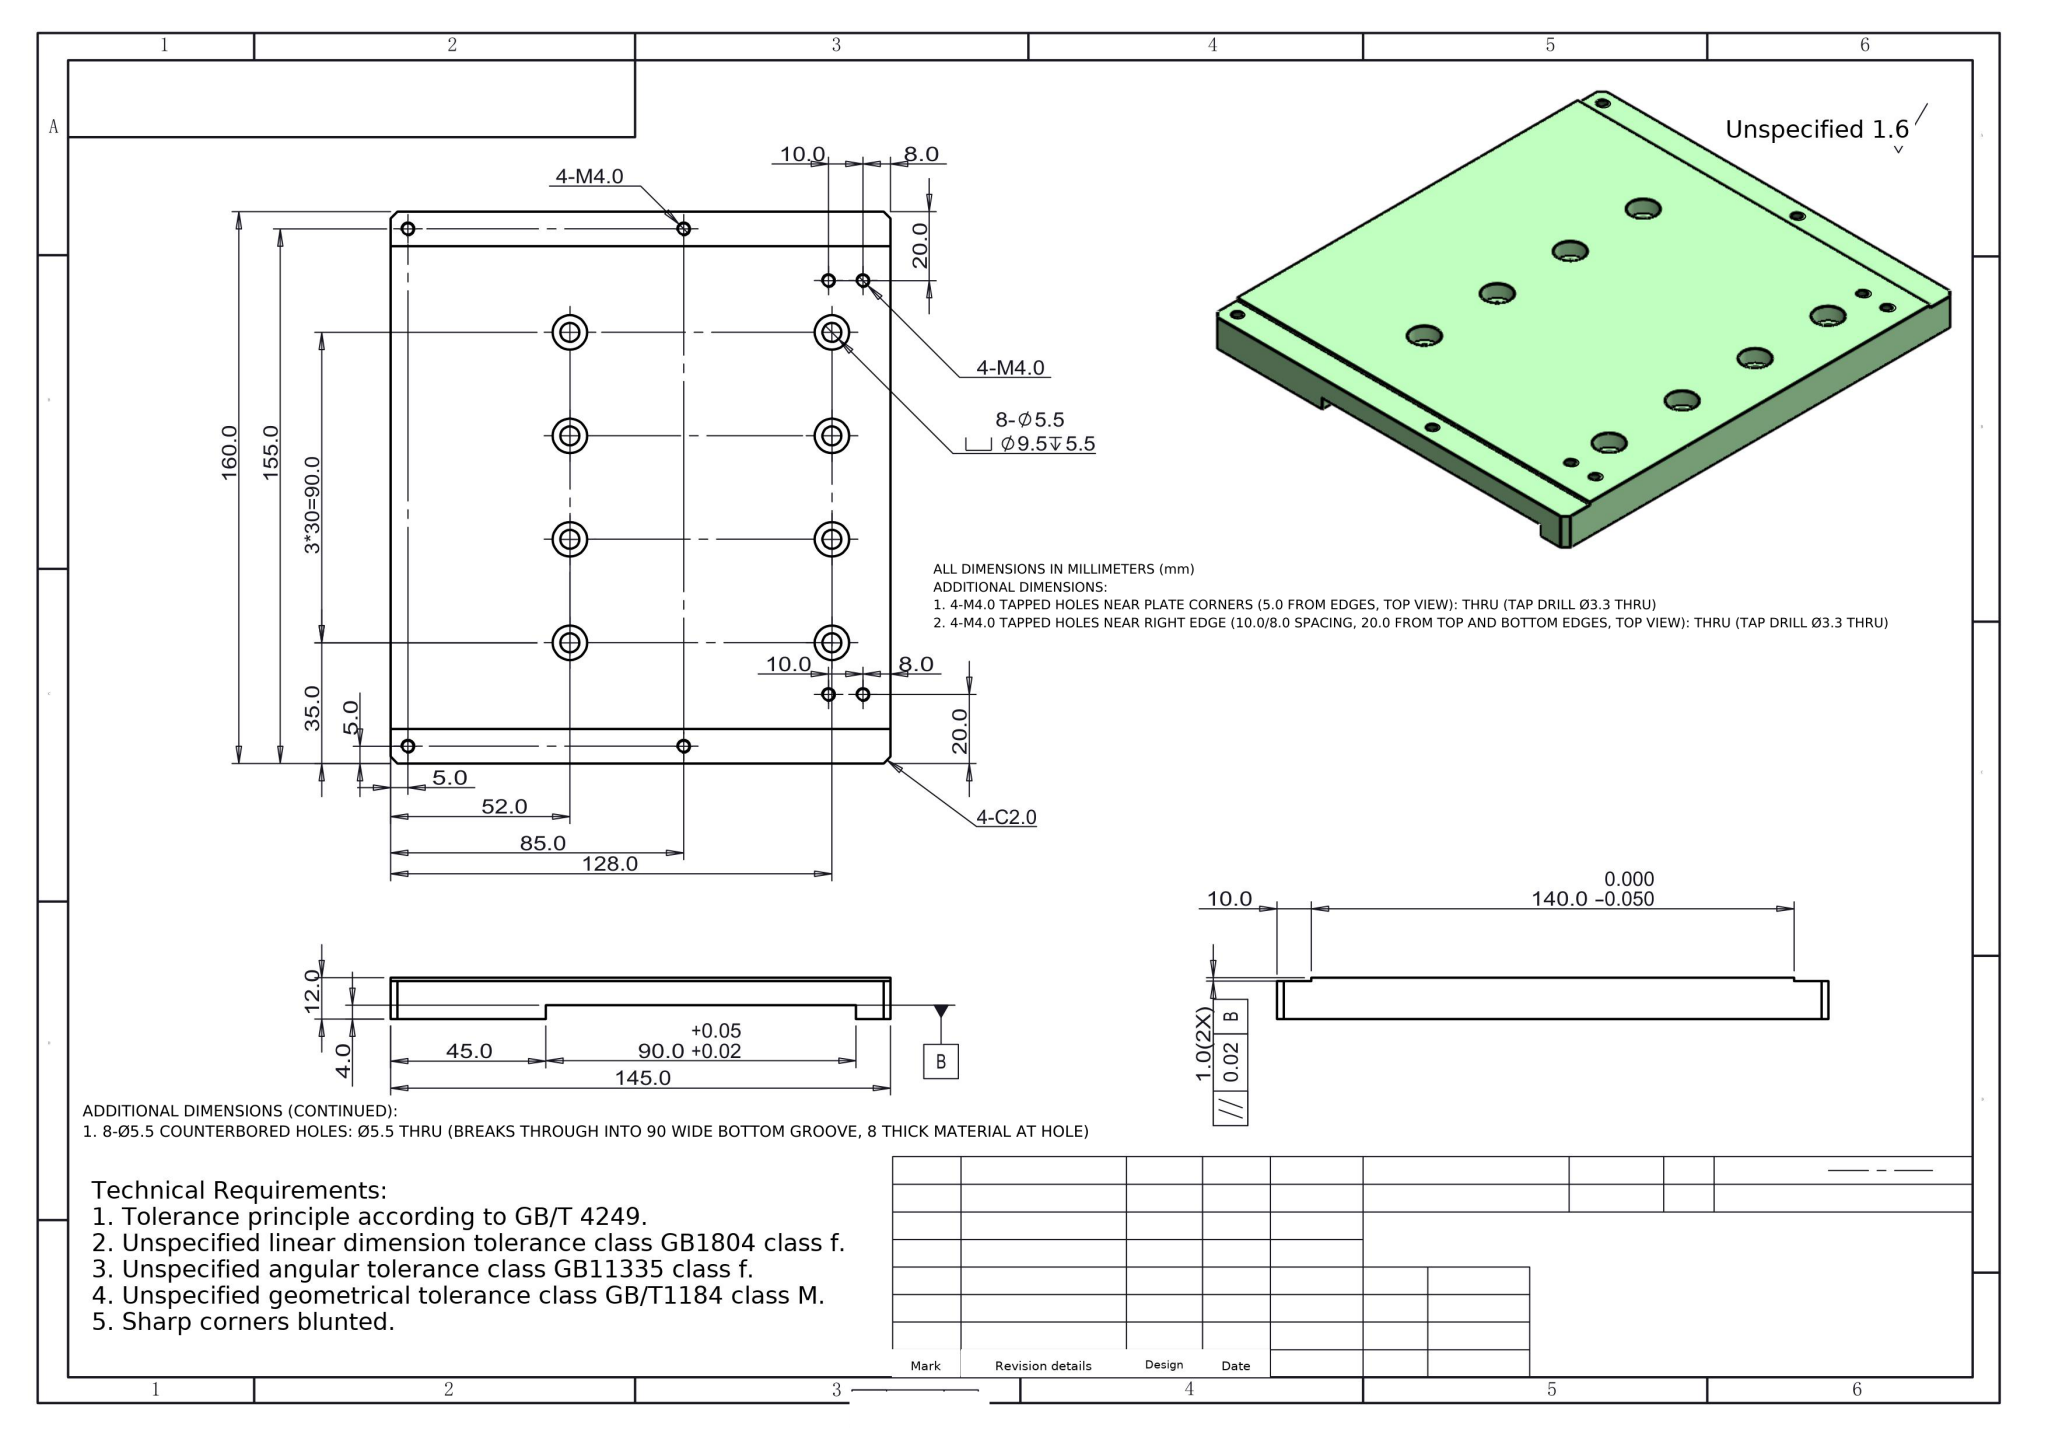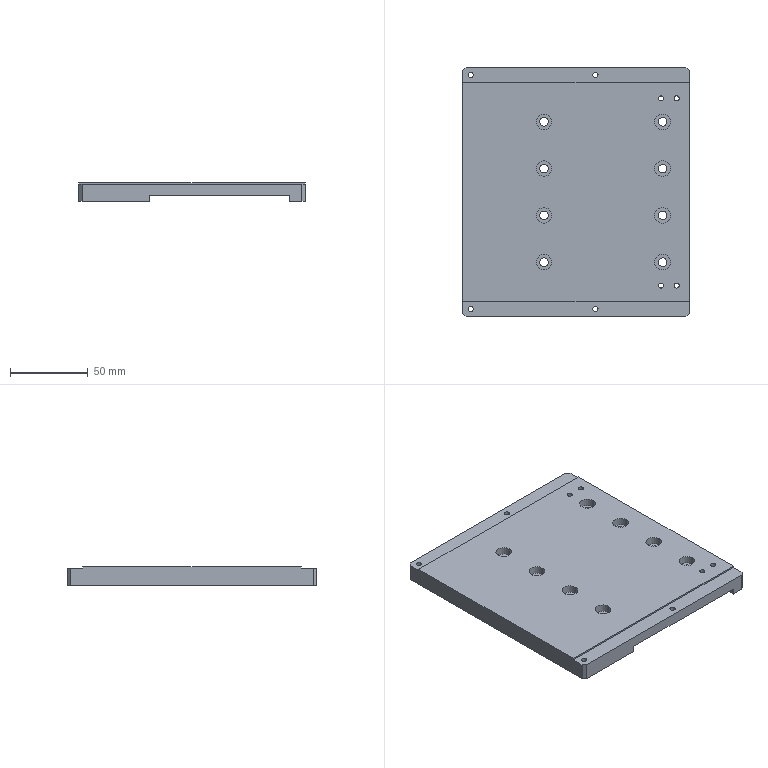Part | NX | mm | 1 solid | 74 faces | box 145 x 160 x 12 mm | volume 213450 mm3 | cylinder 48 | plane 26 | commonest cylinder face diameters 3.3 x16 10 x16 5.5 x16